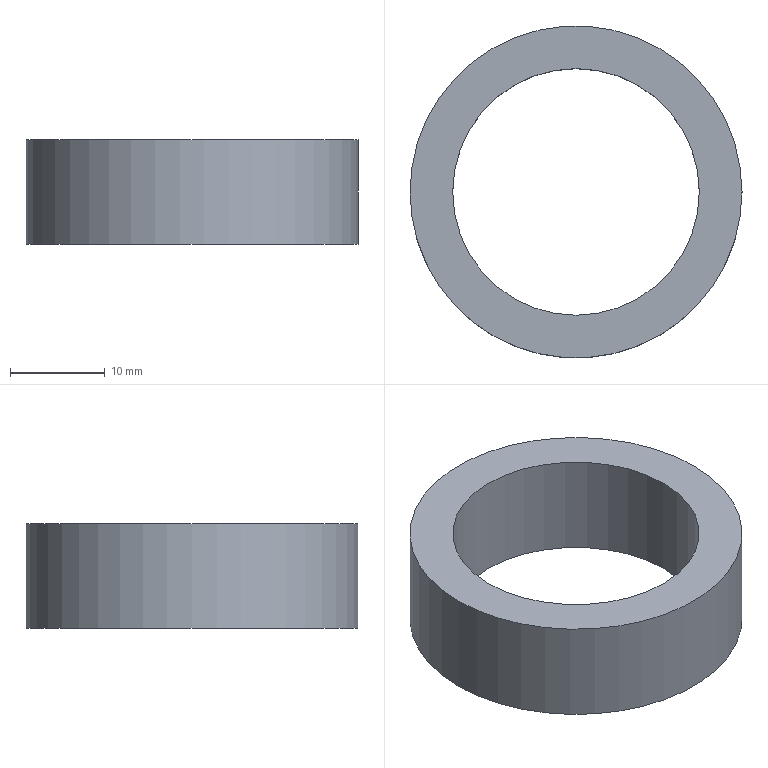Component | NX | SHAFT_SLEEVE | 1 solid | 4 faces | box 35 x 35 x 11 mm | volume 4743 mm3 | cylinder 2 | plane 2 | commonest cylinder face diameters 35 x1 26 x1
STEP:
#1=CARTESIAN_POINT('',(0.,0.,0.));
#2=DIRECTION('',(0.,0.,1.));
#3=DIRECTION('',(1.,0.,0.));
#4=AXIS2_PLACEMENT_3D('',#1,#2,#3);
#5=CARTESIAN_POINT('',(-580.675,308.181,-669.));
#6=VERTEX_POINT('',#5);
#7=CARTESIAN_POINT('',(-598.175,308.181,-669.));
#8=DIRECTION('',(0.,0.,1.));
#9=DIRECTION('',(1.,0.,0.));
#10=AXIS2_PLACEMENT_3D('',#7,#8,#9);
#11=CIRCLE('',#10,17.5);
#12=CARTESIAN_POINT('',(-598.175,308.181,-669.));
#13=DIRECTION('',(0.,0.,-1.));
#14=DIRECTION('',(-1.,0.,0.));
#15=AXIS2_PLACEMENT_3D('',#12,#13,#14);
#16=CYLINDRICAL_SURFACE('',#15,17.5);
#17=CARTESIAN_POINT('',(9.425,0.));
#18=DIRECTION('',(-1.,0.));
#19=VECTOR('',#18,1.);
#20=LINE('',#17,#19);
#21=(GEOMETRIC_REPRESENTATION_CONTEXT(2)PARAMETRIC_REPRESENTATION_CONTEXT()REPRESENTATION_CONTEXT('',''));
#22=DEFINITIONAL_REPRESENTATION('',(#20),#21);
#23=PCURVE('',#16,#22);
#24=CARTESIAN_POINT('',(-598.175,308.181,-669.));
#25=DIRECTION('',(0.,0.,1.));
#26=DIRECTION('',(1.,0.,0.));
#27=AXIS2_PLACEMENT_3D('',#24,#25,#26);
#28=PLANE('',#27);
#29=CARTESIAN_POINT('',(0.,0.));
#30=DIRECTION('',(1.,0.));
#31=AXIS2_PLACEMENT_2D('',#29,#30);
#32=CIRCLE('',#31,17.5);
#33=(GEOMETRIC_REPRESENTATION_CONTEXT(2)PARAMETRIC_REPRESENTATION_CONTEXT()REPRESENTATION_CONTEXT('',''));
#34=DEFINITIONAL_REPRESENTATION('',(#32),#33);
#35=PCURVE('',#28,#34);
#36=SURFACE_CURVE('',#11,(#23,#35),.PCURVE_S1.);
#37=EDGE_CURVE('',#6,#6,#36,.T.);
#38=ORIENTED_EDGE('',*,*,#37,.F.);
#39=CARTESIAN_POINT('',(-580.675,308.181,-680.));
#40=VERTEX_POINT('',#39);
#41=CARTESIAN_POINT('',(-580.675,308.181,-669.));
#42=CARTESIAN_POINT('',(-580.675,308.181,-680.));
#43=B_SPLINE_CURVE_WITH_KNOTS('',1,(#41,#42),.UNSPECIFIED.,.F.,.F.,(2,2),(0.,11.),.PIECEWISE_BEZIER_KNOTS.);
#44=CARTESIAN_POINT('',(9.425,0.));
#45=DIRECTION('',(0.,1.));
#46=VECTOR('',#45,1.);
#47=LINE('',#44,#46);
#48=(GEOMETRIC_REPRESENTATION_CONTEXT(2)PARAMETRIC_REPRESENTATION_CONTEXT()REPRESENTATION_CONTEXT('',''));
#49=DEFINITIONAL_REPRESENTATION('',(#47),#48);
#50=PCURVE('',#16,#49);
#51=CARTESIAN_POINT('',(3.142,0.));
#52=DIRECTION('',(0.,1.));
#53=VECTOR('',#52,1.);
#54=LINE('',#51,#53);
#55=(GEOMETRIC_REPRESENTATION_CONTEXT(2)PARAMETRIC_REPRESENTATION_CONTEXT()REPRESENTATION_CONTEXT('',''));
#56=DEFINITIONAL_REPRESENTATION('',(#54),#55);
#57=PCURVE('',#16,#56);
#58=SEAM_CURVE('',#43,(#50,#57),.PCURVE_S1.);
#59=EDGE_CURVE('',#6,#40,#58,.T.);
#60=ORIENTED_EDGE('',*,*,#59,.T.);
#61=CARTESIAN_POINT('',(-598.175,308.181,-680.));
#62=DIRECTION('',(0.,0.,1.));
#63=DIRECTION('',(1.,0.,0.));
#64=AXIS2_PLACEMENT_3D('',#61,#62,#63);
#65=CIRCLE('',#64,17.5);
#66=CARTESIAN_POINT('',(9.425,11.));
#67=DIRECTION('',(-1.,0.));
#68=VECTOR('',#67,1.);
#69=LINE('',#66,#68);
#70=(GEOMETRIC_REPRESENTATION_CONTEXT(2)PARAMETRIC_REPRESENTATION_CONTEXT()REPRESENTATION_CONTEXT('',''));
#71=DEFINITIONAL_REPRESENTATION('',(#69),#70);
#72=PCURVE('',#16,#71);
#73=CARTESIAN_POINT('',(-598.175,308.181,-680.));
#74=DIRECTION('',(0.,0.,1.));
#75=DIRECTION('',(1.,0.,0.));
#76=AXIS2_PLACEMENT_3D('',#73,#74,#75);
#77=PLANE('',#76);
#78=CARTESIAN_POINT('',(0.,0.));
#79=DIRECTION('',(1.,0.));
#80=AXIS2_PLACEMENT_2D('',#78,#79);
#81=CIRCLE('',#80,17.5);
#82=(GEOMETRIC_REPRESENTATION_CONTEXT(2)PARAMETRIC_REPRESENTATION_CONTEXT()REPRESENTATION_CONTEXT('',''));
#83=DEFINITIONAL_REPRESENTATION('',(#81),#82);
#84=PCURVE('',#77,#83);
#85=SURFACE_CURVE('',#65,(#72,#84),.PCURVE_S1.);
#86=EDGE_CURVE('',#40,#40,#85,.T.);
#87=ORIENTED_EDGE('',*,*,#86,.T.);
#88=ORIENTED_EDGE('',*,*,#59,.F.);
#89=EDGE_LOOP('',(#38,#60,#87,#88));
#90=FACE_BOUND('',#89,.T.);
#91=ADVANCED_FACE('',(#90),#16,.T.);
#92=CARTESIAN_POINT('',(-585.175,308.181,-669.));
#93=VERTEX_POINT('',#92);
#94=CARTESIAN_POINT('',(-598.175,308.181,-669.));
#95=DIRECTION('',(0.,0.,1.));
#96=DIRECTION('',(1.,0.,0.));
#97=AXIS2_PLACEMENT_3D('',#94,#95,#96);
#98=CIRCLE('',#97,13.);
#99=CARTESIAN_POINT('',(-598.175,308.181,-669.));
#100=DIRECTION('',(0.,0.,-1.));
#101=DIRECTION('',(-1.,0.,0.));
#102=AXIS2_PLACEMENT_3D('',#99,#100,#101);
#103=CYLINDRICAL_SURFACE('',#102,13.);
#104=CARTESIAN_POINT('',(9.425,0.));
#105=DIRECTION('',(-1.,0.));
#106=VECTOR('',#105,1.);
#107=LINE('',#104,#106);
#108=(GEOMETRIC_REPRESENTATION_CONTEXT(2)PARAMETRIC_REPRESENTATION_CONTEXT()REPRESENTATION_CONTEXT('',''));
#109=DEFINITIONAL_REPRESENTATION('',(#107),#108);
#110=PCURVE('',#103,#109);
#111=CARTESIAN_POINT('',(0.,0.));
#112=DIRECTION('',(1.,0.));
#113=AXIS2_PLACEMENT_2D('',#111,#112);
#114=CIRCLE('',#113,13.);
#115=(GEOMETRIC_REPRESENTATION_CONTEXT(2)PARAMETRIC_REPRESENTATION_CONTEXT()REPRESENTATION_CONTEXT('',''));
#116=DEFINITIONAL_REPRESENTATION('',(#114),#115);
#117=PCURVE('',#28,#116);
#118=SURFACE_CURVE('',#98,(#110,#117),.PCURVE_S1.);
#119=EDGE_CURVE('',#93,#93,#118,.T.);
#120=ORIENTED_EDGE('',*,*,#119,.F.);
#121=CARTESIAN_POINT('',(-585.175,308.181,-680.));
#122=VERTEX_POINT('',#121);
#123=CARTESIAN_POINT('',(-585.175,308.181,-669.));
#124=CARTESIAN_POINT('',(-585.175,308.181,-680.));
#125=B_SPLINE_CURVE_WITH_KNOTS('',1,(#123,#124),.UNSPECIFIED.,.F.,.F.,(2,2),(0.,11.),.PIECEWISE_BEZIER_KNOTS.);
#126=CARTESIAN_POINT('',(9.425,0.));
#127=DIRECTION('',(0.,1.));
#128=VECTOR('',#127,1.);
#129=LINE('',#126,#128);
#130=(GEOMETRIC_REPRESENTATION_CONTEXT(2)PARAMETRIC_REPRESENTATION_CONTEXT()REPRESENTATION_CONTEXT('',''));
#131=DEFINITIONAL_REPRESENTATION('',(#129),#130);
#132=PCURVE('',#103,#131);
#133=CARTESIAN_POINT('',(3.142,0.));
#134=DIRECTION('',(0.,1.));
#135=VECTOR('',#134,1.);
#136=LINE('',#133,#135);
#137=(GEOMETRIC_REPRESENTATION_CONTEXT(2)PARAMETRIC_REPRESENTATION_CONTEXT()REPRESENTATION_CONTEXT('',''));
#138=DEFINITIONAL_REPRESENTATION('',(#136),#137);
#139=PCURVE('',#103,#138);
#140=SEAM_CURVE('',#125,(#132,#139),.PCURVE_S1.);
#141=EDGE_CURVE('',#93,#122,#140,.T.);
#142=ORIENTED_EDGE('',*,*,#141,.T.);
#143=CARTESIAN_POINT('',(-598.175,308.181,-680.));
#144=DIRECTION('',(0.,0.,1.));
#145=DIRECTION('',(1.,0.,0.));
#146=AXIS2_PLACEMENT_3D('',#143,#144,#145);
#147=CIRCLE('',#146,13.);
#148=CARTESIAN_POINT('',(9.425,11.));
#149=DIRECTION('',(-1.,0.));
#150=VECTOR('',#149,1.);
#151=LINE('',#148,#150);
#152=(GEOMETRIC_REPRESENTATION_CONTEXT(2)PARAMETRIC_REPRESENTATION_CONTEXT()REPRESENTATION_CONTEXT('',''));
#153=DEFINITIONAL_REPRESENTATION('',(#151),#152);
#154=PCURVE('',#103,#153);
#155=CARTESIAN_POINT('',(0.,0.));
#156=DIRECTION('',(1.,0.));
#157=AXIS2_PLACEMENT_2D('',#155,#156);
#158=CIRCLE('',#157,13.);
#159=(GEOMETRIC_REPRESENTATION_CONTEXT(2)PARAMETRIC_REPRESENTATION_CONTEXT()REPRESENTATION_CONTEXT('',''));
#160=DEFINITIONAL_REPRESENTATION('',(#158),#159);
#161=PCURVE('',#77,#160);
#162=SURFACE_CURVE('',#147,(#154,#161),.PCURVE_S1.);
#163=EDGE_CURVE('',#122,#122,#162,.T.);
#164=ORIENTED_EDGE('',*,*,#163,.T.);
#165=ORIENTED_EDGE('',*,*,#141,.F.);
#166=EDGE_LOOP('',(#120,#142,#164,#165));
#167=FACE_BOUND('',#166,.F.);
#168=ADVANCED_FACE('',(#167),#103,.F.);
#169=ORIENTED_EDGE('',*,*,#37,.T.);
#170=EDGE_LOOP('',(#169));
#171=FACE_BOUND('',#170,.T.);
#172=ORIENTED_EDGE('',*,*,#119,.F.);
#173=EDGE_LOOP('',(#172));
#174=FACE_BOUND('',#173,.T.);
#175=ADVANCED_FACE('',(#171,#174),#28,.T.);
#176=ORIENTED_EDGE('',*,*,#86,.F.);
#177=EDGE_LOOP('',(#176));
#178=FACE_BOUND('',#177,.T.);
#179=ORIENTED_EDGE('',*,*,#163,.T.);
#180=EDGE_LOOP('',(#179));
#181=FACE_BOUND('',#180,.T.);
#182=ADVANCED_FACE('',(#178,#181),#77,.F.);
#183=CLOSED_SHELL('',(#91,#168,#175,#182));
#184=MANIFOLD_SOLID_BREP('',#183);
#185=(LENGTH_UNIT()NAMED_UNIT(*)SI_UNIT(.MILLI.,.METRE.));
#186=UNCERTAINTY_MEASURE_WITH_UNIT(LENGTH_MEASURE(0.00001),#185,'','');
#187=(NAMED_UNIT(*)PLANE_ANGLE_UNIT()SI_UNIT($,.RADIAN.));
#188=(NAMED_UNIT(*)SI_UNIT($,.STERADIAN.)SOLID_ANGLE_UNIT());
#189=(GEOMETRIC_REPRESENTATION_CONTEXT(3)GLOBAL_UNCERTAINTY_ASSIGNED_CONTEXT((#186))GLOBAL_UNIT_ASSIGNED_CONTEXT((#185,#187,#188))REPRESENTATION_CONTEXT('',''));
#190=ADVANCED_BREP_SHAPE_REPRESENTATION('',(#4,#184),#189);